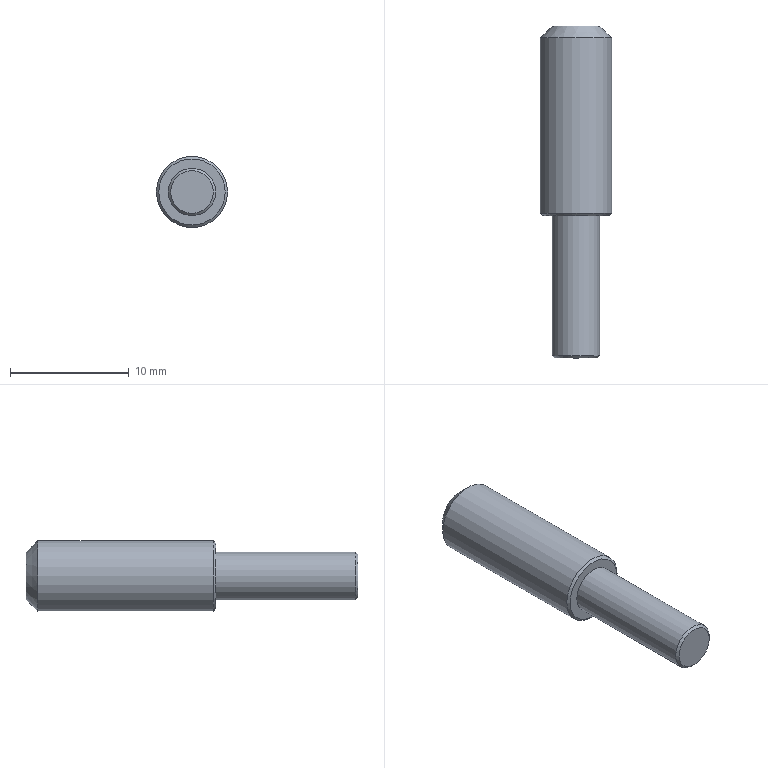Component | NX | SMALL_SHAFT | 1 solid | 8 faces | box 6 x 28 x 6 mm | volume 594 mm3 | plane 3 | cone 3 | cylinder 2 | commonest cylinder face diameters 6 x1 4 x1
STEP:
#1=CARTESIAN_POINT('',(0.,0.,0.));
#2=DIRECTION('',(0.,0.,1.));
#3=DIRECTION('',(1.,0.,0.));
#4=AXIS2_PLACEMENT_3D('',#1,#2,#3);
#5=CARTESIAN_POINT('',(2.8,-30.5,4.5));
#6=VERTEX_POINT('',#5);
#7=CARTESIAN_POINT('',(-0.,-30.5,4.5));
#8=DIRECTION('',(0.,-1.,0.));
#9=DIRECTION('',(1.,0.,0.));
#10=AXIS2_PLACEMENT_3D('',#7,#8,#9);
#11=CIRCLE('',#10,2.8);
#12=CARTESIAN_POINT('',(-0.,-30.5,4.5));
#13=DIRECTION('',(0.,-1.,0.));
#14=DIRECTION('',(1.,0.,0.));
#15=AXIS2_PLACEMENT_3D('',#12,#13,#14);
#16=PLANE('',#15);
#17=CARTESIAN_POINT('',(0.,0.));
#18=DIRECTION('',(1.,0.));
#19=AXIS2_PLACEMENT_2D('',#17,#18);
#20=CIRCLE('',#19,2.8);
#21=(GEOMETRIC_REPRESENTATION_CONTEXT(2)PARAMETRIC_REPRESENTATION_CONTEXT()REPRESENTATION_CONTEXT('',''));
#22=DEFINITIONAL_REPRESENTATION('',(#20),#21);
#23=PCURVE('',#16,#22);
#24=CARTESIAN_POINT('',(-0.,-30.3,4.5));
#25=DIRECTION('',(0.,1.,0.));
#26=DIRECTION('',(-1.,0.,0.));
#27=AXIS2_PLACEMENT_3D('',#24,#25,#26);
#28=CONICAL_SURFACE('',#27,3.,0.7854);
#29=CARTESIAN_POINT('',(9.425,-0.2));
#30=DIRECTION('',(-1.,0.));
#31=VECTOR('',#30,1.);
#32=LINE('',#29,#31);
#33=(GEOMETRIC_REPRESENTATION_CONTEXT(2)PARAMETRIC_REPRESENTATION_CONTEXT()REPRESENTATION_CONTEXT('',''));
#34=DEFINITIONAL_REPRESENTATION('',(#32),#33);
#35=PCURVE('',#28,#34);
#36=SURFACE_CURVE('',#11,(#23,#35),.PCURVE_S1.);
#37=EDGE_CURVE('',#6,#6,#36,.T.);
#38=ORIENTED_EDGE('',*,*,#37,.T.);
#39=EDGE_LOOP('',(#38));
#40=FACE_BOUND('',#39,.T.);
#41=CARTESIAN_POINT('',(2.,-30.5,4.5));
#42=VERTEX_POINT('',#41);
#43=CARTESIAN_POINT('',(-0.,-30.5,4.5));
#44=DIRECTION('',(0.,-1.,0.));
#45=DIRECTION('',(1.,0.,0.));
#46=AXIS2_PLACEMENT_3D('',#43,#44,#45);
#47=CIRCLE('',#46,2.);
#48=CARTESIAN_POINT('',(0.,0.));
#49=DIRECTION('',(1.,0.));
#50=AXIS2_PLACEMENT_2D('',#48,#49);
#51=CIRCLE('',#50,2.);
#52=(GEOMETRIC_REPRESENTATION_CONTEXT(2)PARAMETRIC_REPRESENTATION_CONTEXT()REPRESENTATION_CONTEXT('',''));
#53=DEFINITIONAL_REPRESENTATION('',(#51),#52);
#54=PCURVE('',#16,#53);
#55=CARTESIAN_POINT('',(-0.,-30.5,4.5));
#56=DIRECTION('',(0.,-1.,0.));
#57=DIRECTION('',(1.,0.,0.));
#58=AXIS2_PLACEMENT_3D('',#55,#56,#57);
#59=CYLINDRICAL_SURFACE('',#58,2.);
#60=CARTESIAN_POINT('',(0.,0.));
#61=DIRECTION('',(1.,0.));
#62=VECTOR('',#61,1.);
#63=LINE('',#60,#62);
#64=(GEOMETRIC_REPRESENTATION_CONTEXT(2)PARAMETRIC_REPRESENTATION_CONTEXT()REPRESENTATION_CONTEXT('',''));
#65=DEFINITIONAL_REPRESENTATION('',(#63),#64);
#66=PCURVE('',#59,#65);
#67=SURFACE_CURVE('',#47,(#54,#66),.PCURVE_S1.);
#68=EDGE_CURVE('',#42,#42,#67,.T.);
#69=ORIENTED_EDGE('',*,*,#68,.F.);
#70=EDGE_LOOP('',(#69));
#71=FACE_BOUND('',#70,.T.);
#72=ADVANCED_FACE('',(#40,#71),#16,.T.);
#73=CARTESIAN_POINT('',(-2.,-14.5,4.5));
#74=VERTEX_POINT('',#73);
#75=CARTESIAN_POINT('',(-0.,-14.5,4.5));
#76=DIRECTION('',(0.,1.,0.));
#77=DIRECTION('',(-1.,0.,0.));
#78=AXIS2_PLACEMENT_3D('',#75,#76,#77);
#79=CIRCLE('',#78,2.);
#80=CARTESIAN_POINT('',(-0.,-14.5,4.5));
#81=DIRECTION('',(0.,1.,0.));
#82=DIRECTION('',(-1.,0.,0.));
#83=AXIS2_PLACEMENT_3D('',#80,#81,#82);
#84=PLANE('',#83);
#85=CARTESIAN_POINT('',(0.,0.));
#86=DIRECTION('',(1.,0.));
#87=AXIS2_PLACEMENT_2D('',#85,#86);
#88=CIRCLE('',#87,2.);
#89=(GEOMETRIC_REPRESENTATION_CONTEXT(2)PARAMETRIC_REPRESENTATION_CONTEXT()REPRESENTATION_CONTEXT('',''));
#90=DEFINITIONAL_REPRESENTATION('',(#88),#89);
#91=PCURVE('',#84,#90);
#92=CARTESIAN_POINT('',(-0.,-15.5,4.5));
#93=DIRECTION('',(0.,-1.,0.));
#94=DIRECTION('',(1.,0.,0.));
#95=AXIS2_PLACEMENT_3D('',#92,#93,#94);
#96=CONICAL_SURFACE('',#95,3.,0.7854);
#97=CARTESIAN_POINT('',(9.425,-1.));
#98=DIRECTION('',(-1.,0.));
#99=VECTOR('',#98,1.);
#100=LINE('',#97,#99);
#101=(GEOMETRIC_REPRESENTATION_CONTEXT(2)PARAMETRIC_REPRESENTATION_CONTEXT()REPRESENTATION_CONTEXT('',''));
#102=DEFINITIONAL_REPRESENTATION('',(#100),#101);
#103=PCURVE('',#96,#102);
#104=SURFACE_CURVE('',#79,(#91,#103),.PCURVE_S1.);
#105=EDGE_CURVE('',#74,#74,#104,.T.);
#106=ORIENTED_EDGE('',*,*,#105,.T.);
#107=EDGE_LOOP('',(#106));
#108=FACE_BOUND('',#107,.T.);
#109=ADVANCED_FACE('',(#108),#84,.T.);
#110=CARTESIAN_POINT('',(3.,-30.3,4.5));
#111=VERTEX_POINT('',#110);
#112=CARTESIAN_POINT('',(-0.,-30.3,4.5));
#113=DIRECTION('',(0.,1.,0.));
#114=DIRECTION('',(1.,0.,0.));
#115=AXIS2_PLACEMENT_3D('',#112,#113,#114);
#116=CIRCLE('',#115,3.);
#117=CARTESIAN_POINT('',(-0.,-14.5,4.5));
#118=DIRECTION('',(0.,-1.,0.));
#119=DIRECTION('',(1.,0.,0.));
#120=AXIS2_PLACEMENT_3D('',#117,#118,#119);
#121=CYLINDRICAL_SURFACE('',#120,3.);
#122=CARTESIAN_POINT('',(6.283,15.8));
#123=DIRECTION('',(-1.,0.));
#124=VECTOR('',#123,1.);
#125=LINE('',#122,#124);
#126=(GEOMETRIC_REPRESENTATION_CONTEXT(2)PARAMETRIC_REPRESENTATION_CONTEXT()REPRESENTATION_CONTEXT('',''));
#127=DEFINITIONAL_REPRESENTATION('',(#125),#126);
#128=PCURVE('',#121,#127);
#129=CARTESIAN_POINT('',(3.142,0.));
#130=DIRECTION('',(1.,0.));
#131=VECTOR('',#130,1.);
#132=LINE('',#129,#131);
#133=(GEOMETRIC_REPRESENTATION_CONTEXT(2)PARAMETRIC_REPRESENTATION_CONTEXT()REPRESENTATION_CONTEXT('',''));
#134=DEFINITIONAL_REPRESENTATION('',(#132),#133);
#135=PCURVE('',#28,#134);
#136=SURFACE_CURVE('',#116,(#128,#135),.PCURVE_S1.);
#137=EDGE_CURVE('',#111,#111,#136,.T.);
#138=ORIENTED_EDGE('',*,*,#137,.T.);
#139=CARTESIAN_POINT('',(3.,-15.5,4.5));
#140=VERTEX_POINT('',#139);
#141=CARTESIAN_POINT('',(3.,-15.5,4.5));
#142=CARTESIAN_POINT('',(3.,-30.3,4.5));
#143=B_SPLINE_CURVE_WITH_KNOTS('',1,(#141,#142),.UNSPECIFIED.,.F.,.F.,(2,2),(1.,15.8),.PIECEWISE_BEZIER_KNOTS.);
#144=CARTESIAN_POINT('',(0.,0.));
#145=DIRECTION('',(0.,1.));
#146=VECTOR('',#145,1.);
#147=LINE('',#144,#146);
#148=(GEOMETRIC_REPRESENTATION_CONTEXT(2)PARAMETRIC_REPRESENTATION_CONTEXT()REPRESENTATION_CONTEXT('',''));
#149=DEFINITIONAL_REPRESENTATION('',(#147),#148);
#150=PCURVE('',#121,#149);
#151=CARTESIAN_POINT('',(6.283,0.));
#152=DIRECTION('',(0.,1.));
#153=VECTOR('',#152,1.);
#154=LINE('',#151,#153);
#155=(GEOMETRIC_REPRESENTATION_CONTEXT(2)PARAMETRIC_REPRESENTATION_CONTEXT()REPRESENTATION_CONTEXT('',''));
#156=DEFINITIONAL_REPRESENTATION('',(#154),#155);
#157=PCURVE('',#121,#156);
#158=SEAM_CURVE('',#143,(#150,#157),.PCURVE_S1.);
#159=EDGE_CURVE('',#140,#111,#158,.T.);
#160=ORIENTED_EDGE('',*,*,#159,.F.);
#161=CARTESIAN_POINT('',(-3.,-15.5,4.5));
#162=VERTEX_POINT('',#161);
#163=CARTESIAN_POINT('',(-0.,-15.5,4.5));
#164=DIRECTION('',(0.,-1.,0.));
#165=DIRECTION('',(-1.,0.,0.));
#166=AXIS2_PLACEMENT_3D('',#163,#164,#165);
#167=CIRCLE('',#166,3.);
#168=CARTESIAN_POINT('',(-3.142,1.));
#169=DIRECTION('',(1.,0.));
#170=VECTOR('',#169,1.);
#171=LINE('',#168,#170);
#172=(GEOMETRIC_REPRESENTATION_CONTEXT(2)PARAMETRIC_REPRESENTATION_CONTEXT()REPRESENTATION_CONTEXT('',''));
#173=DEFINITIONAL_REPRESENTATION('',(#171),#172);
#174=PCURVE('',#121,#173);
#175=CARTESIAN_POINT('',(3.142,0.));
#176=DIRECTION('',(1.,0.));
#177=VECTOR('',#176,1.);
#178=LINE('',#175,#177);
#179=(GEOMETRIC_REPRESENTATION_CONTEXT(2)PARAMETRIC_REPRESENTATION_CONTEXT()REPRESENTATION_CONTEXT('',''));
#180=DEFINITIONAL_REPRESENTATION('',(#178),#179);
#181=PCURVE('',#96,#180);
#182=SURFACE_CURVE('',#167,(#174,#181),.PCURVE_S1.);
#183=EDGE_CURVE('',#140,#162,#182,.T.);
#184=ORIENTED_EDGE('',*,*,#183,.T.);
#185=CARTESIAN_POINT('',(-0.,-15.5,4.5));
#186=DIRECTION('',(0.,-1.,0.));
#187=DIRECTION('',(-1.,0.,0.));
#188=AXIS2_PLACEMENT_3D('',#185,#186,#187);
#189=CIRCLE('',#188,3.);
#190=CARTESIAN_POINT('',(3.142,1.));
#191=DIRECTION('',(1.,0.));
#192=VECTOR('',#191,1.);
#193=LINE('',#190,#192);
#194=(GEOMETRIC_REPRESENTATION_CONTEXT(2)PARAMETRIC_REPRESENTATION_CONTEXT()REPRESENTATION_CONTEXT('',''));
#195=DEFINITIONAL_REPRESENTATION('',(#193),#194);
#196=PCURVE('',#121,#195);
#197=CARTESIAN_POINT('',(3.142,0.));
#198=DIRECTION('',(1.,0.));
#199=VECTOR('',#198,1.);
#200=LINE('',#197,#199);
#201=(GEOMETRIC_REPRESENTATION_CONTEXT(2)PARAMETRIC_REPRESENTATION_CONTEXT()REPRESENTATION_CONTEXT('',''));
#202=DEFINITIONAL_REPRESENTATION('',(#200),#201);
#203=PCURVE('',#96,#202);
#204=SURFACE_CURVE('',#189,(#196,#203),.PCURVE_S1.);
#205=EDGE_CURVE('',#162,#140,#204,.T.);
#206=ORIENTED_EDGE('',*,*,#205,.T.);
#207=ORIENTED_EDGE('',*,*,#159,.T.);
#208=EDGE_LOOP('',(#138,#160,#184,#206,#207));
#209=FACE_BOUND('',#208,.T.);
#210=ADVANCED_FACE('',(#209),#121,.T.);
#211=CARTESIAN_POINT('',(1.8,-42.5,4.5));
#212=VERTEX_POINT('',#211);
#213=CARTESIAN_POINT('',(-0.,-42.5,4.5));
#214=DIRECTION('',(0.,-1.,0.));
#215=DIRECTION('',(1.,0.,0.));
#216=AXIS2_PLACEMENT_3D('',#213,#214,#215);
#217=CIRCLE('',#216,1.8);
#218=CARTESIAN_POINT('',(-0.,-42.5,4.5));
#219=DIRECTION('',(0.,-1.,0.));
#220=DIRECTION('',(1.,0.,0.));
#221=AXIS2_PLACEMENT_3D('',#218,#219,#220);
#222=PLANE('',#221);
#223=CARTESIAN_POINT('',(0.,0.));
#224=DIRECTION('',(1.,0.));
#225=AXIS2_PLACEMENT_2D('',#223,#224);
#226=CIRCLE('',#225,1.8);
#227=(GEOMETRIC_REPRESENTATION_CONTEXT(2)PARAMETRIC_REPRESENTATION_CONTEXT()REPRESENTATION_CONTEXT('',''));
#228=DEFINITIONAL_REPRESENTATION('',(#226),#227);
#229=PCURVE('',#222,#228);
#230=CARTESIAN_POINT('',(-0.,-42.5,4.5));
#231=DIRECTION('',(0.,1.,0.));
#232=DIRECTION('',(-1.,0.,0.));
#233=AXIS2_PLACEMENT_3D('',#230,#231,#232);
#234=CONICAL_SURFACE('',#233,1.8,0.7854);
#235=CARTESIAN_POINT('',(9.425,0.));
#236=DIRECTION('',(-1.,0.));
#237=VECTOR('',#236,1.);
#238=LINE('',#235,#237);
#239=(GEOMETRIC_REPRESENTATION_CONTEXT(2)PARAMETRIC_REPRESENTATION_CONTEXT()REPRESENTATION_CONTEXT('',''));
#240=DEFINITIONAL_REPRESENTATION('',(#238),#239);
#241=PCURVE('',#234,#240);
#242=SURFACE_CURVE('',#217,(#229,#241),.PCURVE_S1.);
#243=EDGE_CURVE('',#212,#212,#242,.T.);
#244=ORIENTED_EDGE('',*,*,#243,.T.);
#245=EDGE_LOOP('',(#244));
#246=FACE_BOUND('',#245,.T.);
#247=ADVANCED_FACE('',(#246),#222,.T.);
#248=CARTESIAN_POINT('',(2.,-42.3,4.5));
#249=VERTEX_POINT('',#248);
#250=CARTESIAN_POINT('',(-0.,-42.3,4.5));
#251=DIRECTION('',(0.,1.,0.));
#252=DIRECTION('',(1.,0.,0.));
#253=AXIS2_PLACEMENT_3D('',#250,#251,#252);
#254=CIRCLE('',#253,2.);
#255=CARTESIAN_POINT('',(6.283,11.8));
#256=DIRECTION('',(-1.,0.));
#257=VECTOR('',#256,1.);
#258=LINE('',#255,#257);
#259=(GEOMETRIC_REPRESENTATION_CONTEXT(2)PARAMETRIC_REPRESENTATION_CONTEXT()REPRESENTATION_CONTEXT('',''));
#260=DEFINITIONAL_REPRESENTATION('',(#258),#259);
#261=PCURVE('',#59,#260);
#262=CARTESIAN_POINT('',(3.142,0.2));
#263=DIRECTION('',(1.,0.));
#264=VECTOR('',#263,1.);
#265=LINE('',#262,#264);
#266=(GEOMETRIC_REPRESENTATION_CONTEXT(2)PARAMETRIC_REPRESENTATION_CONTEXT()REPRESENTATION_CONTEXT('',''));
#267=DEFINITIONAL_REPRESENTATION('',(#265),#266);
#268=PCURVE('',#234,#267);
#269=SURFACE_CURVE('',#254,(#261,#268),.PCURVE_S1.);
#270=EDGE_CURVE('',#249,#249,#269,.T.);
#271=ORIENTED_EDGE('',*,*,#270,.T.);
#272=CARTESIAN_POINT('',(2.,-30.5,4.5));
#273=CARTESIAN_POINT('',(2.,-42.3,4.5));
#274=B_SPLINE_CURVE_WITH_KNOTS('',1,(#272,#273),.UNSPECIFIED.,.F.,.F.,(2,2),(0.,11.8),.PIECEWISE_BEZIER_KNOTS.);
#275=CARTESIAN_POINT('',(0.,0.));
#276=DIRECTION('',(0.,1.));
#277=VECTOR('',#276,1.);
#278=LINE('',#275,#277);
#279=(GEOMETRIC_REPRESENTATION_CONTEXT(2)PARAMETRIC_REPRESENTATION_CONTEXT()REPRESENTATION_CONTEXT('',''));
#280=DEFINITIONAL_REPRESENTATION('',(#278),#279);
#281=PCURVE('',#59,#280);
#282=CARTESIAN_POINT('',(6.283,0.));
#283=DIRECTION('',(0.,1.));
#284=VECTOR('',#283,1.);
#285=LINE('',#282,#284);
#286=(GEOMETRIC_REPRESENTATION_CONTEXT(2)PARAMETRIC_REPRESENTATION_CONTEXT()REPRESENTATION_CONTEXT('',''));
#287=DEFINITIONAL_REPRESENTATION('',(#285),#286);
#288=PCURVE('',#59,#287);
#289=SEAM_CURVE('',#274,(#281,#288),.PCURVE_S1.);
#290=EDGE_CURVE('',#42,#249,#289,.T.);
#291=ORIENTED_EDGE('',*,*,#290,.F.);
#292=ORIENTED_EDGE('',*,*,#68,.T.);
#293=ORIENTED_EDGE('',*,*,#290,.T.);
#294=EDGE_LOOP('',(#271,#291,#292,#293));
#295=FACE_BOUND('',#294,.T.);
#296=ADVANCED_FACE('',(#295),#59,.T.);
#297=ORIENTED_EDGE('',*,*,#105,.F.);
#298=CARTESIAN_POINT('',(-2.,-14.5,4.5));
#299=CARTESIAN_POINT('',(-3.,-15.5,4.5));
#300=B_SPLINE_CURVE_WITH_KNOTS('',1,(#298,#299),.UNSPECIFIED.,.F.,.F.,(2,2),(-1.414,0.),.PIECEWISE_BEZIER_KNOTS.);
#301=CARTESIAN_POINT('',(9.425,0.));
#302=DIRECTION('',(0.,1.));
#303=VECTOR('',#302,1.);
#304=LINE('',#301,#303);
#305=(GEOMETRIC_REPRESENTATION_CONTEXT(2)PARAMETRIC_REPRESENTATION_CONTEXT()REPRESENTATION_CONTEXT('',''));
#306=DEFINITIONAL_REPRESENTATION('',(#304),#305);
#307=PCURVE('',#96,#306);
#308=CARTESIAN_POINT('',(3.142,0.));
#309=DIRECTION('',(0.,1.));
#310=VECTOR('',#309,1.);
#311=LINE('',#308,#310);
#312=(GEOMETRIC_REPRESENTATION_CONTEXT(2)PARAMETRIC_REPRESENTATION_CONTEXT()REPRESENTATION_CONTEXT('',''));
#313=DEFINITIONAL_REPRESENTATION('',(#311),#312);
#314=PCURVE('',#96,#313);
#315=SEAM_CURVE('',#300,(#307,#314),.PCURVE_S1.);
#316=EDGE_CURVE('',#74,#162,#315,.T.);
#317=ORIENTED_EDGE('',*,*,#316,.T.);
#318=ORIENTED_EDGE('',*,*,#183,.F.);
#319=ORIENTED_EDGE('',*,*,#205,.F.);
#320=ORIENTED_EDGE('',*,*,#316,.F.);
#321=EDGE_LOOP('',(#297,#317,#318,#319,#320));
#322=FACE_BOUND('',#321,.T.);
#323=ADVANCED_FACE('',(#322),#96,.T.);
#324=ORIENTED_EDGE('',*,*,#270,.F.);
#325=CARTESIAN_POINT('',(1.8,-42.5,4.5));
#326=CARTESIAN_POINT('',(2.,-42.3,4.5));
#327=B_SPLINE_CURVE_WITH_KNOTS('',1,(#325,#326),.UNSPECIFIED.,.F.,.F.,(2,2),(0.,0.2828),.PIECEWISE_BEZIER_KNOTS.);
#328=CARTESIAN_POINT('',(3.142,0.));
#329=DIRECTION('',(0.,1.));
#330=VECTOR('',#329,1.);
#331=LINE('',#328,#330);
#332=(GEOMETRIC_REPRESENTATION_CONTEXT(2)PARAMETRIC_REPRESENTATION_CONTEXT()REPRESENTATION_CONTEXT('',''));
#333=DEFINITIONAL_REPRESENTATION('',(#331),#332);
#334=PCURVE('',#234,#333);
#335=CARTESIAN_POINT('',(9.425,0.));
#336=DIRECTION('',(0.,1.));
#337=VECTOR('',#336,1.);
#338=LINE('',#335,#337);
#339=(GEOMETRIC_REPRESENTATION_CONTEXT(2)PARAMETRIC_REPRESENTATION_CONTEXT()REPRESENTATION_CONTEXT('',''));
#340=DEFINITIONAL_REPRESENTATION('',(#338),#339);
#341=PCURVE('',#234,#340);
#342=SEAM_CURVE('',#327,(#334,#341),.PCURVE_S1.);
#343=EDGE_CURVE('',#212,#249,#342,.T.);
#344=ORIENTED_EDGE('',*,*,#343,.F.);
#345=ORIENTED_EDGE('',*,*,#243,.F.);
#346=ORIENTED_EDGE('',*,*,#343,.T.);
#347=EDGE_LOOP('',(#324,#344,#345,#346));
#348=FACE_BOUND('',#347,.T.);
#349=ADVANCED_FACE('',(#348),#234,.T.);
#350=ORIENTED_EDGE('',*,*,#37,.F.);
#351=CARTESIAN_POINT('',(2.8,-30.5,4.5));
#352=CARTESIAN_POINT('',(3.,-30.3,4.5));
#353=B_SPLINE_CURVE_WITH_KNOTS('',1,(#351,#352),.UNSPECIFIED.,.F.,.F.,(2,2),(-0.2828,0.),.PIECEWISE_BEZIER_KNOTS.);
#354=CARTESIAN_POINT('',(9.425,0.));
#355=DIRECTION('',(0.,1.));
#356=VECTOR('',#355,1.);
#357=LINE('',#354,#356);
#358=(GEOMETRIC_REPRESENTATION_CONTEXT(2)PARAMETRIC_REPRESENTATION_CONTEXT()REPRESENTATION_CONTEXT('',''));
#359=DEFINITIONAL_REPRESENTATION('',(#357),#358);
#360=PCURVE('',#28,#359);
#361=CARTESIAN_POINT('',(3.142,0.));
#362=DIRECTION('',(0.,1.));
#363=VECTOR('',#362,1.);
#364=LINE('',#361,#363);
#365=(GEOMETRIC_REPRESENTATION_CONTEXT(2)PARAMETRIC_REPRESENTATION_CONTEXT()REPRESENTATION_CONTEXT('',''));
#366=DEFINITIONAL_REPRESENTATION('',(#364),#365);
#367=PCURVE('',#28,#366);
#368=SEAM_CURVE('',#353,(#360,#367),.PCURVE_S1.);
#369=EDGE_CURVE('',#6,#111,#368,.T.);
#370=ORIENTED_EDGE('',*,*,#369,.T.);
#371=ORIENTED_EDGE('',*,*,#137,.F.);
#372=ORIENTED_EDGE('',*,*,#369,.F.);
#373=EDGE_LOOP('',(#350,#370,#371,#372));
#374=FACE_BOUND('',#373,.T.);
#375=ADVANCED_FACE('',(#374),#28,.T.);
#376=CLOSED_SHELL('',(#72,#109,#210,#247,#296,#323,#349,#375));
#377=MANIFOLD_SOLID_BREP('',#376);
#378=(LENGTH_UNIT()NAMED_UNIT(*)SI_UNIT(.MILLI.,.METRE.));
#379=UNCERTAINTY_MEASURE_WITH_UNIT(LENGTH_MEASURE(0.00001),#378,'','');
#380=(NAMED_UNIT(*)PLANE_ANGLE_UNIT()SI_UNIT($,.RADIAN.));
#381=(NAMED_UNIT(*)SI_UNIT($,.STERADIAN.)SOLID_ANGLE_UNIT());
#382=(GEOMETRIC_REPRESENTATION_CONTEXT(3)GLOBAL_UNCERTAINTY_ASSIGNED_CONTEXT((#379))GLOBAL_UNIT_ASSIGNED_CONTEXT((#378,#380,#381))REPRESENTATION_CONTEXT('',''));
#383=ADVANCED_BREP_SHAPE_REPRESENTATION('',(#4,#377),#382);